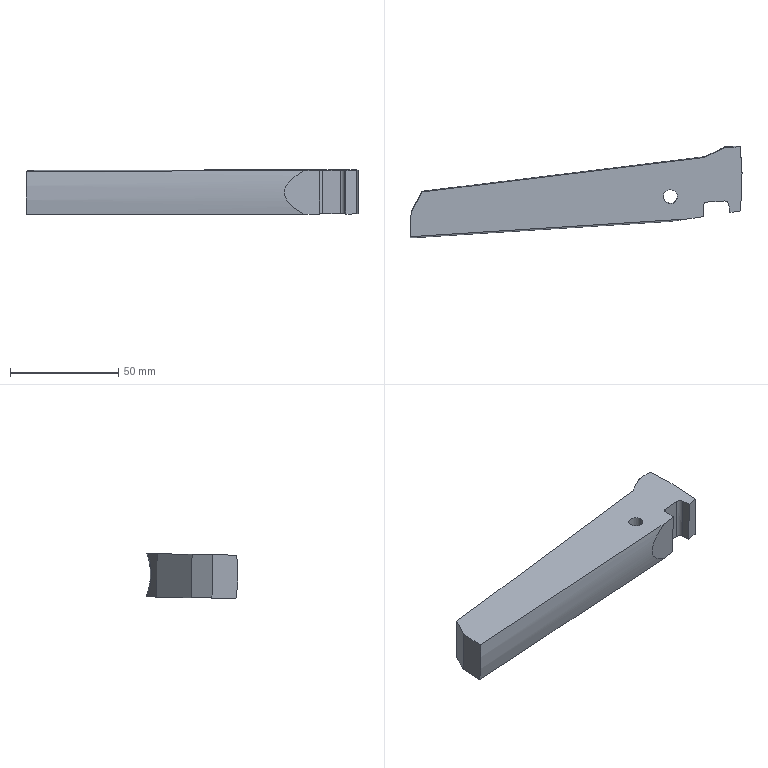Component | SolidWorks | 216InnerTubeAssembly-1_SpringPlate-3 | 1 solid | 21 faces | box 153.4 x 42.53 x 20.74 mm | volume 73490 mm3 | plane 13 | cylinder 6 | cone 2 | commonest cylinder face diameters 6.5 x2 4 x2 65 x1 127 x1 | material Alloy Steel
STEP:
#1=COLOUR_RGB('',0.7922,0.8196,0.9333);
#2=FILL_AREA_STYLE_COLOUR('',#1);
#3=FILL_AREA_STYLE('',(#2));
#4=SURFACE_STYLE_FILL_AREA(#3);
#5=SURFACE_SIDE_STYLE('',(#4));
#6=SURFACE_STYLE_USAGE(.BOTH.,#5);
#7=PRESENTATION_STYLE_ASSIGNMENT((#6));
#8=CARTESIAN_POINT('',(19.681,-0.6175,-0.4049));
#9=VERTEX_POINT('',#8);
#10=CARTESIAN_POINT('',(19.526,-0.6967,-0.01254));
#11=VERTEX_POINT('',#10);
#12=CARTESIAN_POINT('',(19.681,-0.6175,-0.4049));
#13=CARTESIAN_POINT('',(19.659,-0.6283,-0.3776));
#14=CARTESIAN_POINT('',(19.639,-0.6384,-0.3491));
#15=CARTESIAN_POINT('',(19.601,-0.6568,-0.2893));
#16=CARTESIAN_POINT('',(19.585,-0.6651,-0.258));
#17=CARTESIAN_POINT('',(19.564,-0.6758,-0.2081));
#18=CARTESIAN_POINT('',(19.557,-0.679,-0.1911));
#19=CARTESIAN_POINT('',(19.546,-0.6847,-0.1567));
#20=CARTESIAN_POINT('',(19.542,-0.6872,-0.1392));
#21=CARTESIAN_POINT('',(19.534,-0.6914,-0.1038));
#22=CARTESIAN_POINT('',(19.531,-0.6931,-0.08582));
#23=CARTESIAN_POINT('',(19.527,-0.6956,-0.0493));
#24=CARTESIAN_POINT('',(19.526,-0.6964,-0.03081));
#25=CARTESIAN_POINT('',(19.526,-0.6967,-0.01254));
#26=B_SPLINE_CURVE_WITH_KNOTS('',3,(#12,#13,#14,#15,#16,#17,#18,#19,#20,#21,#22,#23,#24,#25),.UNSPECIFIED.,.F.,.F.,(4,2,2,2,2,2,4),(0.00000026,0.002773,0.005546,0.006933,0.00832,0.009706,0.01109),.UNSPECIFIED.);
#27=EDGE_CURVE('',#9,#11,#26,.T.);
#28=ORIENTED_EDGE('',*,*,#27,.T.);
#29=CARTESIAN_POINT('',(19.709,-0.7457,-0.01342));
#30=VERTEX_POINT('',#29);
#31=CARTESIAN_POINT('',(19.921,-0.8026,-0.01444));
#32=DIRECTION('',(0.9659,-0.2588,-0.004647));
#33=VECTOR('',#32,39.37);
#34=LINE('',#31,#33);
#35=EDGE_CURVE('',#11,#30,#34,.T.);
#36=ORIENTED_EDGE('',*,*,#35,.T.);
#37=CARTESIAN_POINT('',(19.702,-0.624,-0.405));
#38=VERTEX_POINT('',#37);
#39=CARTESIAN_POINT('',(19.709,-0.7457,-0.01342));
#40=CARTESIAN_POINT('',(19.709,-0.7432,-0.1538));
#41=CARTESIAN_POINT('',(19.706,-0.7015,-0.2879));
#42=CARTESIAN_POINT('',(19.702,-0.624,-0.405));
#43=(BOUNDED_CURVE()B_SPLINE_CURVE(3,(#39,#40,#41,#42),.UNSPECIFIED.,.F.,.F.)B_SPLINE_CURVE_WITH_KNOTS((4,4),(0.,0.5668),.UNSPECIFIED.)CURVE()GEOMETRIC_REPRESENTATION_ITEM()RATIONAL_B_SPLINE_CURVE((1.,0.9734,0.9734,1.))REPRESENTATION_ITEM(''));
#44=EDGE_CURVE('',#30,#38,#43,.T.);
#45=ORIENTED_EDGE('',*,*,#44,.T.);
#46=CARTESIAN_POINT('',(19.681,-0.6175,-0.4049));
#47=CARTESIAN_POINT('',(19.688,-0.6197,-0.4049));
#48=CARTESIAN_POINT('',(19.695,-0.6218,-0.405));
#49=CARTESIAN_POINT('',(19.702,-0.624,-0.405));
#50=B_SPLINE_CURVE_WITH_KNOTS('',3,(#46,#47,#48,#49),.UNSPECIFIED.,.F.,.F.,(4,4),(0.01645,0.01699),.UNSPECIFIED.);
#51=EDGE_CURVE('',#9,#38,#50,.T.);
#52=ORIENTED_EDGE('',*,*,#51,.F.);
#53=EDGE_LOOP('',(#28,#36,#45,#52));
#54=FACE_OUTER_BOUND('',#53,.T.);
#55=CARTESIAN_POINT('',(19.921,0.00000045,-0.0000253));
#56=DIRECTION('',(1.,-0.,-0.));
#57=DIRECTION('',(-0.,-0.9998,-0.01796));
#58=AXIS2_PLACEMENT_3D('',#55,#56,#57);
#59=CONICAL_SURFACE('',#58,0.8027,0.2618);
#60=ADVANCED_FACE('',(#54),#59,.F.);
#61=CARTESIAN_POINT('',(18.301,-1.536,-0.4214));
#62=VERTEX_POINT('',#61);
#63=CARTESIAN_POINT('',(18.556,-1.52,-0.4211));
#64=VERTEX_POINT('',#63);
#65=CARTESIAN_POINT('',(18.429,-1.528,-0.4212));
#66=DIRECTION('',(-0.,0.01796,-0.9998));
#67=DIRECTION('',(0.998,0.06365,0.001143));
#68=AXIS2_PLACEMENT_3D('',#65,#66,#67);
#69=CIRCLE('',#68,0.128);
#70=EDGE_CURVE('',#62,#64,#69,.T.);
#71=ORIENTED_EDGE('',*,*,#70,.T.);
#72=CARTESIAN_POINT('',(18.556,-1.534,0.3662));
#73=VERTEX_POINT('',#72);
#74=CARTESIAN_POINT('',(18.556,-1.52,-0.4211));
#75=DIRECTION('',(0.,-0.01796,0.9998));
#76=VECTOR('',#75,39.37);
#77=LINE('',#74,#76);
#78=EDGE_CURVE('',#64,#73,#77,.T.);
#79=ORIENTED_EDGE('',*,*,#78,.T.);
#80=CARTESIAN_POINT('',(18.301,-1.55,0.3659));
#81=VERTEX_POINT('',#80);
#82=CARTESIAN_POINT('',(18.429,-1.542,0.366));
#83=DIRECTION('',(-0.,0.01796,-0.9998));
#84=DIRECTION('',(0.998,0.06365,0.001143));
#85=AXIS2_PLACEMENT_3D('',#82,#83,#84);
#86=CIRCLE('',#85,0.128);
#87=EDGE_CURVE('',#81,#73,#86,.T.);
#88=ORIENTED_EDGE('',*,*,#87,.F.);
#89=CARTESIAN_POINT('',(18.301,-1.536,-0.4214));
#90=DIRECTION('',(0.,-0.01796,0.9998));
#91=VECTOR('',#90,39.37);
#92=LINE('',#89,#91);
#93=EDGE_CURVE('',#62,#81,#92,.T.);
#94=ORIENTED_EDGE('',*,*,#93,.F.);
#95=EDGE_LOOP('',(#71,#79,#88,#94));
#96=FACE_OUTER_BOUND('',#95,.T.);
#97=CARTESIAN_POINT('',(18.429,-1.528,-0.4212));
#98=DIRECTION('',(0.,-0.01796,0.9998));
#99=DIRECTION('',(-0.998,-0.06365,-0.001143));
#100=AXIS2_PLACEMENT_3D('',#97,#98,#99);
#101=CYLINDRICAL_SURFACE('',#100,0.128);
#102=ADVANCED_FACE('',(#96),#101,.F.);
#103=ORIENTED_EDGE('',*,*,#70,.F.);
#104=CARTESIAN_POINT('',(18.429,-1.528,-0.4212));
#105=DIRECTION('',(-0.,0.01796,-0.9998));
#106=DIRECTION('',(0.998,0.06365,0.001143));
#107=AXIS2_PLACEMENT_3D('',#104,#105,#106);
#108=CIRCLE('',#107,0.128);
#109=EDGE_CURVE('',#64,#62,#108,.T.);
#110=ORIENTED_EDGE('',*,*,#109,.F.);
#111=EDGE_LOOP('',(#103,#110));
#112=FACE_BOUND('',#111,.T.);
#113=CARTESIAN_POINT('',(19.414,-0.6346,-0.4052));
#114=VERTEX_POINT('',#113);
#115=CARTESIAN_POINT('',(13.611,-1.005,-0.4118));
#116=DIRECTION('',(-0.998,-0.06365,-0.001143));
#117=VECTOR('',#116,39.37);
#118=LINE('',#115,#117);
#119=EDGE_CURVE('',#9,#114,#118,.T.);
#120=ORIENTED_EDGE('',*,*,#119,.F.);
#121=ORIENTED_EDGE('',*,*,#51,.T.);
#122=CARTESIAN_POINT('',(19.732,-1.1,-0.4135));
#123=VERTEX_POINT('',#122);
#124=CARTESIAN_POINT('',(19.701,-0.6129,-0.4048));
#125=DIRECTION('',(0.06366,-0.9978,-0.01792));
#126=VECTOR('',#125,39.37);
#127=LINE('',#124,#126);
#128=EDGE_CURVE('',#38,#123,#127,.T.);
#129=ORIENTED_EDGE('',*,*,#128,.T.);
#130=CARTESIAN_POINT('',(19.708,-1.786,-0.4259));
#131=VERTEX_POINT('',#130);
#132=CARTESIAN_POINT('',(19.732,-1.1,-0.4135));
#133=DIRECTION('',(-0.0357,-0.9992,-0.01794));
#134=VECTOR('',#133,39.37);
#135=LINE('',#132,#134);
#136=EDGE_CURVE('',#123,#131,#135,.T.);
#137=ORIENTED_EDGE('',*,*,#136,.T.);
#138=CARTESIAN_POINT('',(19.512,-1.816,-0.4264));
#139=VERTEX_POINT('',#138);
#140=CARTESIAN_POINT('',(19.708,-1.786,-0.4259));
#141=DIRECTION('',(-0.9886,-0.1504,-0.0027));
#142=VECTOR('',#141,39.37);
#143=LINE('',#140,#142);
#144=EDGE_CURVE('',#131,#139,#143,.T.);
#145=ORIENTED_EDGE('',*,*,#144,.T.);
#146=CARTESIAN_POINT('',(19.49,-1.671,-0.4238));
#147=VERTEX_POINT('',#146);
#148=CARTESIAN_POINT('',(19.512,-1.816,-0.4264));
#149=DIRECTION('',(-0.1504,0.9885,0.01775));
#150=VECTOR('',#149,39.37);
#151=LINE('',#148,#150);
#152=EDGE_CURVE('',#139,#147,#151,.T.);
#153=ORIENTED_EDGE('',*,*,#152,.T.);
#154=CARTESIAN_POINT('',(19.407,-1.604,-0.4226));
#155=VERTEX_POINT('',#154);
#156=CARTESIAN_POINT('',(19.412,-1.683,-0.424));
#157=DIRECTION('',(0.,-0.01796,0.9998));
#158=DIRECTION('',(0.998,0.06365,0.001143));
#159=AXIS2_PLACEMENT_3D('',#156,#157,#158);
#160=CIRCLE('',#159,0.07874);
#161=EDGE_CURVE('',#147,#155,#160,.T.);
#162=ORIENTED_EDGE('',*,*,#161,.T.);
#163=CARTESIAN_POINT('',(19.093,-1.624,-0.423));
#164=VERTEX_POINT('',#163);
#165=CARTESIAN_POINT('',(19.093,-1.624,-0.423));
#166=DIRECTION('',(-0.998,-0.06365,-0.001143));
#167=VECTOR('',#166,39.37);
#168=LINE('',#165,#167);
#169=EDGE_CURVE('',#155,#164,#168,.T.);
#170=ORIENTED_EDGE('',*,*,#169,.T.);
#171=CARTESIAN_POINT('',(19.032,-1.66,-0.4236));
#172=VERTEX_POINT('',#171);
#173=CARTESIAN_POINT('',(19.098,-1.703,-0.4244));
#174=DIRECTION('',(0.,-0.01796,0.9998));
#175=DIRECTION('',(0.998,0.06365,0.001143));
#176=AXIS2_PLACEMENT_3D('',#173,#174,#175);
#177=CIRCLE('',#176,0.07874);
#178=EDGE_CURVE('',#164,#172,#177,.T.);
#179=ORIENTED_EDGE('',*,*,#178,.T.);
#180=CARTESIAN_POINT('',(19.027,-1.888,-0.4277));
#181=VERTEX_POINT('',#180);
#182=CARTESIAN_POINT('',(19.032,-1.66,-0.4236));
#183=DIRECTION('',(-0.02356,-0.9996,-0.01795));
#184=VECTOR('',#183,39.37);
#185=LINE('',#182,#184);
#186=EDGE_CURVE('',#172,#181,#185,.T.);
#187=ORIENTED_EDGE('',*,*,#186,.T.);
#188=CARTESIAN_POINT('',(18.748,-1.931,-0.4285));
#189=VERTEX_POINT('',#188);
#190=CARTESIAN_POINT('',(19.027,-1.888,-0.4277));
#191=DIRECTION('',(-0.9886,-0.1504,-0.0027));
#192=VECTOR('',#191,39.37);
#193=LINE('',#190,#192);
#194=EDGE_CURVE('',#181,#189,#193,.T.);
#195=ORIENTED_EDGE('',*,*,#194,.T.);
#196=CARTESIAN_POINT('',(13.694,-2.253,-0.4343));
#197=VERTEX_POINT('',#196);
#198=CARTESIAN_POINT('',(13.691,-2.253,-0.4343));
#199=DIRECTION('',(-0.998,-0.06365,-0.001143));
#200=VECTOR('',#199,39.37);
#201=LINE('',#198,#200);
#202=EDGE_CURVE('',#189,#197,#201,.T.);
#203=ORIENTED_EDGE('',*,*,#202,.T.);
#204=CARTESIAN_POINT('',(13.714,-1.817,-0.4264));
#205=VERTEX_POINT('',#204);
#206=CARTESIAN_POINT('',(13.693,-2.284,-0.4348));
#207=DIRECTION('',(0.04445,0.9989,0.01794));
#208=VECTOR('',#207,39.37);
#209=LINE('',#206,#208);
#210=EDGE_CURVE('',#197,#205,#209,.T.);
#211=ORIENTED_EDGE('',*,*,#210,.T.);
#212=CARTESIAN_POINT('',(13.909,-1.441,-0.4197));
#213=VERTEX_POINT('',#212);
#214=CARTESIAN_POINT('',(13.714,-1.817,-0.4264));
#215=DIRECTION('',(0.461,0.8872,0.01593));
#216=VECTOR('',#215,39.37);
#217=LINE('',#214,#216);
#218=EDGE_CURVE('',#205,#213,#217,.T.);
#219=ORIENTED_EDGE('',*,*,#218,.T.);
#220=CARTESIAN_POINT('',(19.054,-0.8118,-0.4084));
#221=VERTEX_POINT('',#220);
#222=CARTESIAN_POINT('',(13.909,-1.441,-0.4197));
#223=DIRECTION('',(0.9926,0.1214,0.00218));
#224=VECTOR('',#223,39.37);
#225=LINE('',#222,#224);
#226=EDGE_CURVE('',#213,#221,#225,.T.);
#227=ORIENTED_EDGE('',*,*,#226,.T.);
#228=CARTESIAN_POINT('',(19.422,-0.6307,-0.4051));
#229=DIRECTION('',(0.8972,0.4416,0.007931));
#230=VECTOR('',#229,39.37);
#231=LINE('',#228,#230);
#232=EDGE_CURVE('',#221,#114,#231,.T.);
#233=ORIENTED_EDGE('',*,*,#232,.T.);
#234=EDGE_LOOP('',(#120,#121,#129,#137,#145,#153,#162,#170,#179,#187,#195,#203,#211,#219,#227,#233));
#235=FACE_OUTER_BOUND('',#234,.T.);
#236=CARTESIAN_POINT('',(19.098,-1.703,-0.4244));
#237=DIRECTION('',(-0.,0.01796,-0.9998));
#238=DIRECTION('',(0.998,0.06365,0.001143));
#239=AXIS2_PLACEMENT_3D('',#236,#237,#238);
#240=PLANE('',#239);
#241=ADVANCED_FACE('',(#112,#235),#240,.T.);
#242=ORIENTED_EDGE('',*,*,#87,.T.);
#243=CARTESIAN_POINT('',(18.429,-1.542,0.366));
#244=DIRECTION('',(-0.,0.01796,-0.9998));
#245=DIRECTION('',(0.998,0.06365,0.001143));
#246=AXIS2_PLACEMENT_3D('',#243,#244,#245);
#247=CIRCLE('',#246,0.128);
#248=EDGE_CURVE('',#73,#81,#247,.T.);
#249=ORIENTED_EDGE('',*,*,#248,.T.);
#250=EDGE_LOOP('',(#242,#249));
#251=FACE_BOUND('',#250,.T.);
#252=CARTESIAN_POINT('',(19.681,-0.6317,0.3824));
#253=VERTEX_POINT('',#252);
#254=CARTESIAN_POINT('',(19.702,-0.6381,0.3823));
#255=VERTEX_POINT('',#254);
#256=CARTESIAN_POINT('',(19.681,-0.6317,0.3824));
#257=CARTESIAN_POINT('',(19.688,-0.6338,0.3824));
#258=CARTESIAN_POINT('',(19.695,-0.636,0.3823));
#259=CARTESIAN_POINT('',(19.702,-0.6381,0.3823));
#260=B_SPLINE_CURVE_WITH_KNOTS('',3,(#256,#257,#258,#259),.UNSPECIFIED.,.F.,.F.,(4,4),(0.01645,0.01699),.UNSPECIFIED.);
#261=EDGE_CURVE('',#253,#255,#260,.T.);
#262=ORIENTED_EDGE('',*,*,#261,.F.);
#263=CARTESIAN_POINT('',(19.414,-0.6487,0.3821));
#264=VERTEX_POINT('',#263);
#265=CARTESIAN_POINT('',(13.611,-1.019,0.3754));
#266=DIRECTION('',(-0.998,-0.06365,-0.001143));
#267=VECTOR('',#266,39.37);
#268=LINE('',#265,#267);
#269=EDGE_CURVE('',#253,#264,#268,.T.);
#270=ORIENTED_EDGE('',*,*,#269,.T.);
#271=CARTESIAN_POINT('',(19.054,-0.8259,0.3789));
#272=VERTEX_POINT('',#271);
#273=CARTESIAN_POINT('',(19.422,-0.6449,0.3822));
#274=DIRECTION('',(0.8972,0.4416,0.007931));
#275=VECTOR('',#274,39.37);
#276=LINE('',#273,#275);
#277=EDGE_CURVE('',#272,#264,#276,.T.);
#278=ORIENTED_EDGE('',*,*,#277,.F.);
#279=CARTESIAN_POINT('',(13.909,-1.455,0.3676));
#280=VERTEX_POINT('',#279);
#281=CARTESIAN_POINT('',(13.909,-1.455,0.3676));
#282=DIRECTION('',(0.9926,0.1214,0.00218));
#283=VECTOR('',#282,39.37);
#284=LINE('',#281,#283);
#285=EDGE_CURVE('',#280,#272,#284,.T.);
#286=ORIENTED_EDGE('',*,*,#285,.F.);
#287=CARTESIAN_POINT('',(13.714,-1.831,0.3609));
#288=VERTEX_POINT('',#287);
#289=CARTESIAN_POINT('',(13.714,-1.831,0.3609));
#290=DIRECTION('',(0.461,0.8872,0.01593));
#291=VECTOR('',#290,39.37);
#292=LINE('',#289,#291);
#293=EDGE_CURVE('',#288,#280,#292,.T.);
#294=ORIENTED_EDGE('',*,*,#293,.F.);
#295=CARTESIAN_POINT('',(13.694,-2.267,0.353));
#296=VERTEX_POINT('',#295);
#297=CARTESIAN_POINT('',(13.693,-2.299,0.3525));
#298=DIRECTION('',(0.04445,0.9989,0.01794));
#299=VECTOR('',#298,39.37);
#300=LINE('',#297,#299);
#301=EDGE_CURVE('',#296,#288,#300,.T.);
#302=ORIENTED_EDGE('',*,*,#301,.F.);
#303=CARTESIAN_POINT('',(18.748,-1.945,0.3588));
#304=VERTEX_POINT('',#303);
#305=CARTESIAN_POINT('',(13.691,-2.267,0.353));
#306=DIRECTION('',(-0.998,-0.06365,-0.001143));
#307=VECTOR('',#306,39.37);
#308=LINE('',#305,#307);
#309=EDGE_CURVE('',#304,#296,#308,.T.);
#310=ORIENTED_EDGE('',*,*,#309,.F.);
#311=CARTESIAN_POINT('',(19.027,-1.903,0.3596));
#312=VERTEX_POINT('',#311);
#313=CARTESIAN_POINT('',(19.027,-1.903,0.3596));
#314=DIRECTION('',(-0.9886,-0.1504,-0.0027));
#315=VECTOR('',#314,39.37);
#316=LINE('',#313,#315);
#317=EDGE_CURVE('',#312,#304,#316,.T.);
#318=ORIENTED_EDGE('',*,*,#317,.F.);
#319=CARTESIAN_POINT('',(19.032,-1.674,0.3637));
#320=VERTEX_POINT('',#319);
#321=CARTESIAN_POINT('',(19.032,-1.674,0.3637));
#322=DIRECTION('',(-0.02356,-0.9996,-0.01795));
#323=VECTOR('',#322,39.37);
#324=LINE('',#321,#323);
#325=EDGE_CURVE('',#320,#312,#324,.T.);
#326=ORIENTED_EDGE('',*,*,#325,.F.);
#327=CARTESIAN_POINT('',(19.093,-1.639,0.3643));
#328=VERTEX_POINT('',#327);
#329=CARTESIAN_POINT('',(19.098,-1.717,0.3629));
#330=DIRECTION('',(0.,-0.01796,0.9998));
#331=DIRECTION('',(0.998,0.06365,0.001143));
#332=AXIS2_PLACEMENT_3D('',#329,#330,#331);
#333=CIRCLE('',#332,0.07874);
#334=EDGE_CURVE('',#328,#320,#333,.T.);
#335=ORIENTED_EDGE('',*,*,#334,.F.);
#336=CARTESIAN_POINT('',(19.407,-1.619,0.3647));
#337=VERTEX_POINT('',#336);
#338=CARTESIAN_POINT('',(19.093,-1.639,0.3643));
#339=DIRECTION('',(-0.998,-0.06365,-0.001143));
#340=VECTOR('',#339,39.37);
#341=LINE('',#338,#340);
#342=EDGE_CURVE('',#337,#328,#341,.T.);
#343=ORIENTED_EDGE('',*,*,#342,.F.);
#344=CARTESIAN_POINT('',(19.49,-1.685,0.3635));
#345=VERTEX_POINT('',#344);
#346=CARTESIAN_POINT('',(19.412,-1.697,0.3633));
#347=DIRECTION('',(0.,-0.01796,0.9998));
#348=DIRECTION('',(0.998,0.06365,0.001143));
#349=AXIS2_PLACEMENT_3D('',#346,#347,#348);
#350=CIRCLE('',#349,0.07874);
#351=EDGE_CURVE('',#345,#337,#350,.T.);
#352=ORIENTED_EDGE('',*,*,#351,.F.);
#353=CARTESIAN_POINT('',(19.512,-1.83,0.3609));
#354=VERTEX_POINT('',#353);
#355=CARTESIAN_POINT('',(19.512,-1.83,0.3609));
#356=DIRECTION('',(-0.1504,0.9885,0.01775));
#357=VECTOR('',#356,39.37);
#358=LINE('',#355,#357);
#359=EDGE_CURVE('',#354,#345,#358,.T.);
#360=ORIENTED_EDGE('',*,*,#359,.F.);
#361=CARTESIAN_POINT('',(19.708,-1.8,0.3614));
#362=VERTEX_POINT('',#361);
#363=CARTESIAN_POINT('',(19.708,-1.8,0.3614));
#364=DIRECTION('',(-0.9886,-0.1504,-0.0027));
#365=VECTOR('',#364,39.37);
#366=LINE('',#363,#365);
#367=EDGE_CURVE('',#362,#354,#366,.T.);
#368=ORIENTED_EDGE('',*,*,#367,.F.);
#369=CARTESIAN_POINT('',(19.732,-1.114,0.3737));
#370=VERTEX_POINT('',#369);
#371=CARTESIAN_POINT('',(19.732,-1.114,0.3737));
#372=DIRECTION('',(-0.0357,-0.9992,-0.01794));
#373=VECTOR('',#372,39.37);
#374=LINE('',#371,#373);
#375=EDGE_CURVE('',#370,#362,#374,.T.);
#376=ORIENTED_EDGE('',*,*,#375,.F.);
#377=CARTESIAN_POINT('',(19.701,-0.6271,0.3825));
#378=DIRECTION('',(0.06366,-0.9978,-0.01792));
#379=VECTOR('',#378,39.37);
#380=LINE('',#377,#379);
#381=EDGE_CURVE('',#255,#370,#380,.T.);
#382=ORIENTED_EDGE('',*,*,#381,.F.);
#383=EDGE_LOOP('',(#262,#270,#278,#286,#294,#302,#310,#318,#326,#335,#343,#352,#360,#368,#376,#382));
#384=FACE_OUTER_BOUND('',#383,.T.);
#385=CARTESIAN_POINT('',(19.098,-1.717,0.3629));
#386=DIRECTION('',(-0.,0.01796,-0.9998));
#387=DIRECTION('',(0.998,0.06365,0.001143));
#388=AXIS2_PLACEMENT_3D('',#385,#386,#387);
#389=PLANE('',#388);
#390=ADVANCED_FACE('',(#251,#384),#389,.F.);
#391=ORIENTED_EDGE('',*,*,#27,.F.);
#392=ORIENTED_EDGE('',*,*,#119,.T.);
#393=CARTESIAN_POINT('',(19.414,-0.6487,0.3821));
#394=CARTESIAN_POINT('',(19.219,-0.7401,0.1223));
#395=CARTESIAN_POINT('',(19.219,-0.7352,-0.1489));
#396=CARTESIAN_POINT('',(19.414,-0.6346,-0.4052));
#397=(BOUNDED_CURVE()B_SPLINE_CURVE(3,(#393,#394,#395,#396),.UNSPECIFIED.,.F.,.F.)B_SPLINE_CURVE_WITH_KNOTS((4,4),(2.829,3.454),.UNSPECIFIED.)CURVE()GEOMETRIC_REPRESENTATION_ITEM()RATIONAL_B_SPLINE_CURVE((1.,0.9677,0.9677,1.))REPRESENTATION_ITEM(''));
#398=EDGE_CURVE('',#264,#114,#397,.T.);
#399=ORIENTED_EDGE('',*,*,#398,.F.);
#400=ORIENTED_EDGE('',*,*,#269,.F.);
#401=CARTESIAN_POINT('',(19.526,-0.6967,-0.01254));
#402=CARTESIAN_POINT('',(19.526,-0.6973,0.02399));
#403=CARTESIAN_POINT('',(19.53,-0.6962,0.06015));
#404=CARTESIAN_POINT('',(19.541,-0.6918,0.1139));
#405=CARTESIAN_POINT('',(19.546,-0.69,0.1317));
#406=CARTESIAN_POINT('',(19.557,-0.6855,0.1663));
#407=CARTESIAN_POINT('',(19.563,-0.6829,0.1832));
#408=CARTESIAN_POINT('',(19.584,-0.6741,0.2328));
#409=CARTESIAN_POINT('',(19.601,-0.667,0.2646));
#410=CARTESIAN_POINT('',(19.638,-0.6506,0.3257));
#411=CARTESIAN_POINT('',(19.659,-0.6415,0.3547));
#412=CARTESIAN_POINT('',(19.681,-0.6317,0.3824));
#413=B_SPLINE_CURVE_WITH_KNOTS('',3,(#401,#402,#403,#404,#405,#406,#407,#408,#409,#410,#411,#412),.UNSPECIFIED.,.F.,.F.,(4,2,2,2,2,4),(0.01109,0.01386,0.01525,0.01664,0.01941,0.02218),.UNSPECIFIED.);
#414=EDGE_CURVE('',#11,#253,#413,.T.);
#415=ORIENTED_EDGE('',*,*,#414,.F.);
#416=EDGE_LOOP('',(#391,#392,#399,#400,#415));
#417=FACE_OUTER_BOUND('',#416,.T.);
#418=CARTESIAN_POINT('',(13.534,0.2031,0.003622));
#419=DIRECTION('',(0.998,0.06365,0.001143));
#420=DIRECTION('',(0.,-0.01796,0.9998));
#421=AXIS2_PLACEMENT_3D('',#418,#419,#420);
#422=CYLINDRICAL_SURFACE('',#421,1.28);
#423=ADVANCED_FACE('',(#417),#422,.F.);
#424=CARTESIAN_POINT('',(18.748,-1.931,-0.4285));
#425=CARTESIAN_POINT('',(18.275,-2.007,-0.1684));
#426=CARTESIAN_POINT('',(18.275,-2.012,0.0962));
#427=CARTESIAN_POINT('',(18.748,-1.945,0.3588));
#428=(BOUNDED_CURVE()B_SPLINE_CURVE(3,(#424,#425,#426,#427),.UNSPECIFIED.,.F.,.T.)B_SPLINE_CURVE_WITH_KNOTS((4,4),(2.983,3.3),.UNSPECIFIED.)CURVE()GEOMETRIC_REPRESENTATION_ITEM()RATIONAL_B_SPLINE_CURVE((1.,0.9917,0.9917,1.))REPRESENTATION_ITEM(''));
#429=EDGE_CURVE('',#189,#304,#428,.T.);
#430=ORIENTED_EDGE('',*,*,#429,.F.);
#431=ORIENTED_EDGE('',*,*,#194,.F.);
#432=CARTESIAN_POINT('',(19.027,-1.888,-0.4277));
#433=DIRECTION('',(0.,-0.01796,0.9998));
#434=VECTOR('',#433,39.37);
#435=LINE('',#432,#434);
#436=EDGE_CURVE('',#181,#312,#435,.T.);
#437=ORIENTED_EDGE('',*,*,#436,.T.);
#438=ORIENTED_EDGE('',*,*,#317,.T.);
#439=EDGE_LOOP('',(#430,#431,#437,#438));
#440=FACE_OUTER_BOUND('',#439,.T.);
#441=CARTESIAN_POINT('',(19.027,-1.888,-0.4277));
#442=DIRECTION('',(-0.1504,0.9885,0.01775));
#443=DIRECTION('',(0.9886,0.1504,0.0027));
#444=AXIS2_PLACEMENT_3D('',#441,#442,#443);
#445=PLANE('',#444);
#446=ADVANCED_FACE('',(#440),#445,.F.);
#447=CARTESIAN_POINT('',(13.694,-2.267,0.353));
#448=CARTESIAN_POINT('',(13.692,-2.304,0.09095));
#449=CARTESIAN_POINT('',(13.692,-2.3,-0.1737));
#450=CARTESIAN_POINT('',(13.694,-2.253,-0.4343));
#451=(BOUNDED_CURVE()B_SPLINE_CURVE(3,(#447,#448,#449,#450),.UNSPECIFIED.,.F.,.T.)B_SPLINE_CURVE_WITH_KNOTS((4,4),(2.983,3.3),.UNSPECIFIED.)CURVE()GEOMETRIC_REPRESENTATION_ITEM()RATIONAL_B_SPLINE_CURVE((1.,0.9917,0.9917,1.))REPRESENTATION_ITEM(''));
#452=EDGE_CURVE('',#296,#197,#451,.T.);
#453=ORIENTED_EDGE('',*,*,#452,.F.);
#454=ORIENTED_EDGE('',*,*,#301,.T.);
#455=CARTESIAN_POINT('',(13.714,-1.817,-0.4264));
#456=DIRECTION('',(0.,-0.01796,0.9998));
#457=VECTOR('',#456,39.37);
#458=LINE('',#455,#457);
#459=EDGE_CURVE('',#205,#288,#458,.T.);
#460=ORIENTED_EDGE('',*,*,#459,.F.);
#461=ORIENTED_EDGE('',*,*,#210,.F.);
#462=EDGE_LOOP('',(#453,#454,#460,#461));
#463=FACE_OUTER_BOUND('',#462,.T.);
#464=CARTESIAN_POINT('',(13.693,-2.284,-0.4348));
#465=DIRECTION('',(0.999,-0.04445,-0.0007982));
#466=DIRECTION('',(-0.04445,-0.9989,-0.01794));
#467=AXIS2_PLACEMENT_3D('',#464,#465,#466);
#468=PLANE('',#467);
#469=ADVANCED_FACE('',(#463),#468,.F.);
#470=ORIENTED_EDGE('',*,*,#334,.T.);
#471=CARTESIAN_POINT('',(19.032,-1.66,-0.4236));
#472=DIRECTION('',(0.,-0.01796,0.9998));
#473=VECTOR('',#472,39.37);
#474=LINE('',#471,#473);
#475=EDGE_CURVE('',#172,#320,#474,.T.);
#476=ORIENTED_EDGE('',*,*,#475,.F.);
#477=ORIENTED_EDGE('',*,*,#178,.F.);
#478=CARTESIAN_POINT('',(19.093,-1.624,-0.423));
#479=DIRECTION('',(0.,-0.01796,0.9998));
#480=VECTOR('',#479,39.37);
#481=LINE('',#478,#480);
#482=EDGE_CURVE('',#164,#328,#481,.T.);
#483=ORIENTED_EDGE('',*,*,#482,.T.);
#484=EDGE_LOOP('',(#470,#476,#477,#483));
#485=FACE_OUTER_BOUND('',#484,.T.);
#486=CARTESIAN_POINT('',(19.098,-1.703,-0.4244));
#487=DIRECTION('',(0.,-0.01796,0.9998));
#488=DIRECTION('',(-0.998,-0.06365,-0.001143));
#489=AXIS2_PLACEMENT_3D('',#486,#487,#488);
#490=CYLINDRICAL_SURFACE('',#489,0.07874);
#491=ADVANCED_FACE('',(#485),#490,.F.);
#492=ORIENTED_EDGE('',*,*,#325,.T.);
#493=ORIENTED_EDGE('',*,*,#436,.F.);
#494=ORIENTED_EDGE('',*,*,#186,.F.);
#495=ORIENTED_EDGE('',*,*,#475,.T.);
#496=EDGE_LOOP('',(#492,#493,#494,#495));
#497=FACE_OUTER_BOUND('',#496,.T.);
#498=CARTESIAN_POINT('',(19.032,-1.66,-0.4236));
#499=DIRECTION('',(-0.9997,0.02356,0.0004231));
#500=DIRECTION('',(0.02356,0.9996,0.01795));
#501=AXIS2_PLACEMENT_3D('',#498,#499,#500);
#502=PLANE('',#501);
#503=ADVANCED_FACE('',(#497),#502,.F.);
#504=ORIENTED_EDGE('',*,*,#293,.T.);
#505=CARTESIAN_POINT('',(13.909,-1.441,-0.4197));
#506=DIRECTION('',(0.,-0.01796,0.9998));
#507=VECTOR('',#506,39.37);
#508=LINE('',#505,#507);
#509=EDGE_CURVE('',#213,#280,#508,.T.);
#510=ORIENTED_EDGE('',*,*,#509,.F.);
#511=ORIENTED_EDGE('',*,*,#218,.F.);
#512=ORIENTED_EDGE('',*,*,#459,.T.);
#513=EDGE_LOOP('',(#504,#510,#511,#512));
#514=FACE_OUTER_BOUND('',#513,.T.);
#515=CARTESIAN_POINT('',(13.714,-1.817,-0.4264));
#516=DIRECTION('',(0.8874,-0.4609,-0.008278));
#517=DIRECTION('',(-0.461,-0.8872,-0.01593));
#518=AXIS2_PLACEMENT_3D('',#515,#516,#517);
#519=PLANE('',#518);
#520=ADVANCED_FACE('',(#514),#519,.F.);
#521=ORIENTED_EDGE('',*,*,#285,.T.);
#522=CARTESIAN_POINT('',(19.054,-0.8118,-0.4084));
#523=DIRECTION('',(0.,-0.01796,0.9998));
#524=VECTOR('',#523,39.37);
#525=LINE('',#522,#524);
#526=EDGE_CURVE('',#221,#272,#525,.T.);
#527=ORIENTED_EDGE('',*,*,#526,.F.);
#528=ORIENTED_EDGE('',*,*,#226,.F.);
#529=ORIENTED_EDGE('',*,*,#509,.T.);
#530=EDGE_LOOP('',(#521,#527,#528,#529));
#531=FACE_OUTER_BOUND('',#530,.T.);
#532=CARTESIAN_POINT('',(13.909,-1.441,-0.4197));
#533=DIRECTION('',(0.1214,-0.9924,-0.01782));
#534=DIRECTION('',(-0.9926,-0.1214,-0.00218));
#535=AXIS2_PLACEMENT_3D('',#532,#533,#534);
#536=PLANE('',#535);
#537=ADVANCED_FACE('',(#531),#536,.F.);
#538=ORIENTED_EDGE('',*,*,#277,.T.);
#539=ORIENTED_EDGE('',*,*,#398,.T.);
#540=ORIENTED_EDGE('',*,*,#232,.F.);
#541=ORIENTED_EDGE('',*,*,#526,.T.);
#542=EDGE_LOOP('',(#538,#539,#540,#541));
#543=FACE_OUTER_BOUND('',#542,.T.);
#544=CARTESIAN_POINT('',(19.422,-0.6307,-0.4051));
#545=DIRECTION('',(0.4417,-0.897,-0.01611));
#546=DIRECTION('',(-0.8972,-0.4416,-0.007931));
#547=AXIS2_PLACEMENT_3D('',#544,#545,#546);
#548=PLANE('',#547);
#549=ADVANCED_FACE('',(#543),#548,.F.);
#550=CARTESIAN_POINT('',(19.702,-0.6381,0.3823));
#551=CARTESIAN_POINT('',(19.706,-0.7114,0.2625));
#552=CARTESIAN_POINT('',(19.709,-0.7482,0.127));
#553=CARTESIAN_POINT('',(19.709,-0.7457,-0.01342));
#554=(BOUNDED_CURVE()B_SPLINE_CURVE(3,(#550,#551,#552,#553),.UNSPECIFIED.,.F.,.T.)B_SPLINE_CURVE_WITH_KNOTS((4,4),(5.716,6.283),.UNSPECIFIED.)CURVE()GEOMETRIC_REPRESENTATION_ITEM()RATIONAL_B_SPLINE_CURVE((1.,0.9734,0.9734,1.))REPRESENTATION_ITEM(''));
#555=EDGE_CURVE('',#255,#30,#554,.T.);
#556=ORIENTED_EDGE('',*,*,#555,.F.);
#557=ORIENTED_EDGE('',*,*,#381,.T.);
#558=CARTESIAN_POINT('',(19.732,-1.1,-0.4135));
#559=DIRECTION('',(0.,-0.01796,0.9998));
#560=VECTOR('',#559,39.37);
#561=LINE('',#558,#560);
#562=EDGE_CURVE('',#123,#370,#561,.T.);
#563=ORIENTED_EDGE('',*,*,#562,.F.);
#564=ORIENTED_EDGE('',*,*,#128,.F.);
#565=ORIENTED_EDGE('',*,*,#44,.F.);
#566=EDGE_LOOP('',(#556,#557,#563,#564,#565));
#567=FACE_OUTER_BOUND('',#566,.T.);
#568=CARTESIAN_POINT('',(19.701,-0.6129,-0.4048));
#569=DIRECTION('',(-0.998,-0.06365,-0.001143));
#570=DIRECTION('',(-0.,0.01796,-0.9998));
#571=AXIS2_PLACEMENT_3D('',#568,#569,#570);
#572=PLANE('',#571);
#573=ADVANCED_FACE('',(#567),#572,.F.);
#574=ORIENTED_EDGE('',*,*,#375,.T.);
#575=CARTESIAN_POINT('',(19.708,-1.786,-0.4259));
#576=DIRECTION('',(0.,-0.01796,0.9998));
#577=VECTOR('',#576,39.37);
#578=LINE('',#575,#577);
#579=EDGE_CURVE('',#131,#362,#578,.T.);
#580=ORIENTED_EDGE('',*,*,#579,.F.);
#581=ORIENTED_EDGE('',*,*,#136,.F.);
#582=ORIENTED_EDGE('',*,*,#562,.T.);
#583=EDGE_LOOP('',(#574,#580,#581,#582));
#584=FACE_OUTER_BOUND('',#583,.T.);
#585=CARTESIAN_POINT('',(19.732,-1.1,-0.4135));
#586=DIRECTION('',(-0.9994,0.03569,0.000641));
#587=DIRECTION('',(0.0357,0.9992,0.01794));
#588=AXIS2_PLACEMENT_3D('',#585,#586,#587);
#589=PLANE('',#588);
#590=ADVANCED_FACE('',(#584),#589,.F.);
#591=ORIENTED_EDGE('',*,*,#367,.T.);
#592=CARTESIAN_POINT('',(19.512,-1.816,-0.4264));
#593=DIRECTION('',(0.,-0.01796,0.9998));
#594=VECTOR('',#593,39.37);
#595=LINE('',#592,#594);
#596=EDGE_CURVE('',#139,#354,#595,.T.);
#597=ORIENTED_EDGE('',*,*,#596,.F.);
#598=ORIENTED_EDGE('',*,*,#144,.F.);
#599=ORIENTED_EDGE('',*,*,#579,.T.);
#600=EDGE_LOOP('',(#591,#597,#598,#599));
#601=FACE_OUTER_BOUND('',#600,.T.);
#602=CARTESIAN_POINT('',(19.708,-1.786,-0.4259));
#603=DIRECTION('',(-0.1504,0.9885,0.01775));
#604=DIRECTION('',(0.9886,0.1504,0.0027));
#605=AXIS2_PLACEMENT_3D('',#602,#603,#604);
#606=PLANE('',#605);
#607=ADVANCED_FACE('',(#601),#606,.F.);
#608=ORIENTED_EDGE('',*,*,#359,.T.);
#609=CARTESIAN_POINT('',(19.49,-1.671,-0.4238));
#610=DIRECTION('',(0.,-0.01796,0.9998));
#611=VECTOR('',#610,39.37);
#612=LINE('',#609,#611);
#613=EDGE_CURVE('',#147,#345,#612,.T.);
#614=ORIENTED_EDGE('',*,*,#613,.F.);
#615=ORIENTED_EDGE('',*,*,#152,.F.);
#616=ORIENTED_EDGE('',*,*,#596,.T.);
#617=EDGE_LOOP('',(#608,#614,#615,#616));
#618=FACE_OUTER_BOUND('',#617,.T.);
#619=CARTESIAN_POINT('',(19.512,-1.816,-0.4264));
#620=DIRECTION('',(0.9886,0.1504,0.0027));
#621=DIRECTION('',(0.1504,-0.9885,-0.01775));
#622=AXIS2_PLACEMENT_3D('',#619,#620,#621);
#623=PLANE('',#622);
#624=ADVANCED_FACE('',(#618),#623,.F.);
#625=ORIENTED_EDGE('',*,*,#351,.T.);
#626=CARTESIAN_POINT('',(19.407,-1.604,-0.4226));
#627=DIRECTION('',(0.,-0.01796,0.9998));
#628=VECTOR('',#627,39.37);
#629=LINE('',#626,#628);
#630=EDGE_CURVE('',#155,#337,#629,.T.);
#631=ORIENTED_EDGE('',*,*,#630,.F.);
#632=ORIENTED_EDGE('',*,*,#161,.F.);
#633=ORIENTED_EDGE('',*,*,#613,.T.);
#634=EDGE_LOOP('',(#625,#631,#632,#633));
#635=FACE_OUTER_BOUND('',#634,.T.);
#636=CARTESIAN_POINT('',(19.412,-1.683,-0.424));
#637=DIRECTION('',(0.,-0.01796,0.9998));
#638=DIRECTION('',(-0.998,-0.06365,-0.001143));
#639=AXIS2_PLACEMENT_3D('',#636,#637,#638);
#640=CYLINDRICAL_SURFACE('',#639,0.07874);
#641=ADVANCED_FACE('',(#635),#640,.F.);
#642=ORIENTED_EDGE('',*,*,#342,.T.);
#643=ORIENTED_EDGE('',*,*,#482,.F.);
#644=ORIENTED_EDGE('',*,*,#169,.F.);
#645=ORIENTED_EDGE('',*,*,#630,.T.);
#646=EDGE_LOOP('',(#642,#643,#644,#645));
#647=FACE_OUTER_BOUND('',#646,.T.);
#648=CARTESIAN_POINT('',(19.093,-1.624,-0.423));
#649=DIRECTION('',(-0.06366,0.9978,0.01792));
#650=DIRECTION('',(0.,-0.01796,0.9998));
#651=AXIS2_PLACEMENT_3D('',#648,#649,#650);
#652=PLANE('',#651);
#653=ADVANCED_FACE('',(#647),#652,.F.);
#654=ORIENTED_EDGE('',*,*,#78,.F.);
#655=ORIENTED_EDGE('',*,*,#109,.T.);
#656=ORIENTED_EDGE('',*,*,#93,.T.);
#657=ORIENTED_EDGE('',*,*,#248,.F.);
#658=EDGE_LOOP('',(#654,#655,#656,#657));
#659=FACE_OUTER_BOUND('',#658,.T.);
#660=CARTESIAN_POINT('',(18.429,-1.528,-0.4212));
#661=DIRECTION('',(0.,-0.01796,0.9998));
#662=DIRECTION('',(-0.998,-0.06365,-0.001143));
#663=AXIS2_PLACEMENT_3D('',#660,#661,#662);
#664=CYLINDRICAL_SURFACE('',#663,0.128);
#665=ADVANCED_FACE('',(#659),#664,.F.);
#666=ORIENTED_EDGE('',*,*,#309,.T.);
#667=ORIENTED_EDGE('',*,*,#452,.T.);
#668=ORIENTED_EDGE('',*,*,#202,.F.);
#669=ORIENTED_EDGE('',*,*,#429,.T.);
#670=EDGE_LOOP('',(#666,#667,#668,#669));
#671=FACE_OUTER_BOUND('',#670,.T.);
#672=CARTESIAN_POINT('',(13.534,0.2031,0.003622));
#673=DIRECTION('',(0.998,0.06365,0.001143));
#674=DIRECTION('',(0.,-0.01796,0.9998));
#675=AXIS2_PLACEMENT_3D('',#672,#673,#674);
#676=CYLINDRICAL_SURFACE('',#675,2.5);
#677=ADVANCED_FACE('',(#671),#676,.T.);
#678=ORIENTED_EDGE('',*,*,#35,.F.);
#679=ORIENTED_EDGE('',*,*,#414,.T.);
#680=ORIENTED_EDGE('',*,*,#261,.T.);
#681=ORIENTED_EDGE('',*,*,#555,.T.);
#682=EDGE_LOOP('',(#678,#679,#680,#681));
#683=FACE_OUTER_BOUND('',#682,.T.);
#684=CARTESIAN_POINT('',(19.921,0.00000045,-0.0000253));
#685=DIRECTION('',(1.,-0.,-0.));
#686=DIRECTION('',(-0.,-0.9998,-0.01796));
#687=AXIS2_PLACEMENT_3D('',#684,#685,#686);
#688=CONICAL_SURFACE('',#687,0.8027,0.2618);
#689=ADVANCED_FACE('',(#683),#688,.F.);
#690=CLOSED_SHELL('',(#60,#102,#241,#390,#423,#446,#469,#491,#503,#520,#537,#549,#573,#590,#607,#624,#641,#653,#665,#677,#689));
#691=MANIFOLD_SOLID_BREP('',#690);
#692=STYLED_ITEM('',(#7),#691);
#693=(LENGTH_UNIT()NAMED_UNIT(*)SI_UNIT($,.METRE.));
#694=LENGTH_MEASURE_WITH_UNIT(LENGTH_MEASURE(0.0254),#693);
#695=DIMENSIONAL_EXPONENTS(1.,0.,0.,0.,0.,0.,0.);
#696=(CONVERSION_BASED_UNIT('',#694)LENGTH_UNIT()NAMED_UNIT(#695));
#697=UNCERTAINTY_MEASURE_WITH_UNIT(LENGTH_MEASURE(0.00001),#696,'','');
#698=(NAMED_UNIT(*)PLANE_ANGLE_UNIT()SI_UNIT($,.RADIAN.));
#699=(NAMED_UNIT(*)SI_UNIT($,.STERADIAN.)SOLID_ANGLE_UNIT());
#700=(GEOMETRIC_REPRESENTATION_CONTEXT(3)GLOBAL_UNCERTAINTY_ASSIGNED_CONTEXT((#697))GLOBAL_UNIT_ASSIGNED_CONTEXT((#696,#698,#699))REPRESENTATION_CONTEXT('',''));
#701=MECHANICAL_DESIGN_GEOMETRIC_PRESENTATION_REPRESENTATION('',(#692),#700);
#702=PRESENTATION_LAYER_ASSIGNMENT('','',(#692));
#703=CARTESIAN_POINT('',(0.,0.,0.));
#704=DIRECTION('',(0.,0.,1.));
#705=DIRECTION('',(1.,0.,0.));
#706=AXIS2_PLACEMENT_3D('',#703,#704,#705);
#707=(LENGTH_UNIT()NAMED_UNIT(*)SI_UNIT($,.METRE.));
#708=LENGTH_MEASURE_WITH_UNIT(LENGTH_MEASURE(0.0254),#707);
#709=DIMENSIONAL_EXPONENTS(1.,0.,0.,0.,0.,0.,0.);
#710=(CONVERSION_BASED_UNIT('',#708)LENGTH_UNIT()NAMED_UNIT(#709));
#711=UNCERTAINTY_MEASURE_WITH_UNIT(LENGTH_MEASURE(0.00001),#710,'','');
#712=(NAMED_UNIT(*)PLANE_ANGLE_UNIT()SI_UNIT($,.RADIAN.));
#713=(NAMED_UNIT(*)SI_UNIT($,.STERADIAN.)SOLID_ANGLE_UNIT());
#714=(GEOMETRIC_REPRESENTATION_CONTEXT(3)GLOBAL_UNCERTAINTY_ASSIGNED_CONTEXT((#711))GLOBAL_UNIT_ASSIGNED_CONTEXT((#710,#712,#713))REPRESENTATION_CONTEXT('',''));
#715=ADVANCED_BREP_SHAPE_REPRESENTATION('',(#691,#706),#714);